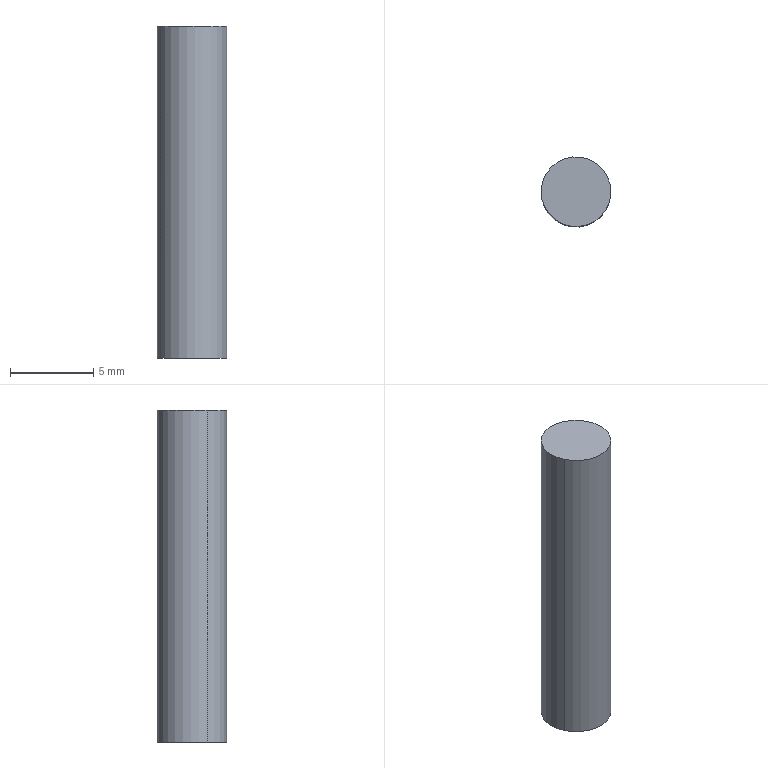Component | SolidWorks | OuterBagStorageAssembly-1_Copy_of_Part1-1 | 1 solid | 4 faces | box 4.2 x 4.2 x 20 mm | volume 277 mm3 | cylinder 2 | plane 2 | commonest cylinder face diameters 4.2 x2
build123d program:
from build123d import *

# Parameters (mm, degrees)
SKETCH1_R           = 2.1
BOSS_EXTRUDE1_DEPTH = 20


with BuildPart() as part:
    # Sketch1 → Boss-Extrude1 (new body)
    with BuildSketch(Plane.XY):
        Circle(SKETCH1_R)
    extrude(amount=BOSS_EXTRUDE1_DEPTH)


solid = part.part

# Placed as in the assembly
solid = solid.moved(Location((-354.296, 148.158, 404.536), (0, 0, 0)))
STEP:
#1=COLOUR_RGB('',0.7922,0.8196,0.9333);
#2=FILL_AREA_STYLE_COLOUR('',#1);
#3=FILL_AREA_STYLE('',(#2));
#4=SURFACE_STYLE_FILL_AREA(#3);
#5=SURFACE_SIDE_STYLE('',(#4));
#6=SURFACE_STYLE_USAGE(.BOTH.,#5);
#7=PRESENTATION_STYLE_ASSIGNMENT((#6));
#8=CARTESIAN_POINT('',(-14.023,5.797,15.927));
#9=VERTEX_POINT('',#8);
#10=CARTESIAN_POINT('',(-13.874,5.869,15.927));
#11=VERTEX_POINT('',#10);
#12=CARTESIAN_POINT('',(-13.949,5.833,15.927));
#13=DIRECTION('',(0.,0.,-1.));
#14=DIRECTION('',(-0.9002,-0.4355,0.));
#15=AXIS2_PLACEMENT_3D('',#12,#13,#14);
#16=CIRCLE('',#15,0.08268);
#17=EDGE_CURVE('',#9,#11,#16,.T.);
#18=ORIENTED_EDGE('',*,*,#17,.F.);
#19=CARTESIAN_POINT('',(-14.023,5.797,16.714));
#20=VERTEX_POINT('',#19);
#21=CARTESIAN_POINT('',(-14.023,5.797,15.927));
#22=DIRECTION('',(-0.,-0.,1.));
#23=VECTOR('',#22,39.37);
#24=LINE('',#21,#23);
#25=EDGE_CURVE('',#9,#20,#24,.T.);
#26=ORIENTED_EDGE('',*,*,#25,.T.);
#27=CARTESIAN_POINT('',(-13.874,5.869,16.714));
#28=VERTEX_POINT('',#27);
#29=CARTESIAN_POINT('',(-13.949,5.833,16.714));
#30=DIRECTION('',(0.,0.,-1.));
#31=DIRECTION('',(-0.9002,-0.4355,0.));
#32=AXIS2_PLACEMENT_3D('',#29,#30,#31);
#33=CIRCLE('',#32,0.08268);
#34=EDGE_CURVE('',#20,#28,#33,.T.);
#35=ORIENTED_EDGE('',*,*,#34,.T.);
#36=CARTESIAN_POINT('',(-13.874,5.869,15.927));
#37=DIRECTION('',(-0.,-0.,1.));
#38=VECTOR('',#37,39.37);
#39=LINE('',#36,#38);
#40=EDGE_CURVE('',#11,#28,#39,.T.);
#41=ORIENTED_EDGE('',*,*,#40,.F.);
#42=EDGE_LOOP('',(#18,#26,#35,#41));
#43=FACE_OUTER_BOUND('',#42,.T.);
#44=CARTESIAN_POINT('',(-13.949,5.833,15.927));
#45=DIRECTION('',(-0.,-0.,1.));
#46=DIRECTION('',(0.9002,0.4355,0.));
#47=AXIS2_PLACEMENT_3D('',#44,#45,#46);
#48=CYLINDRICAL_SURFACE('',#47,0.08268);
#49=ADVANCED_FACE('',(#43),#48,.T.);
#50=ORIENTED_EDGE('',*,*,#25,.F.);
#51=CARTESIAN_POINT('',(-13.949,5.833,15.927));
#52=DIRECTION('',(0.,0.,-1.));
#53=DIRECTION('',(-0.9002,-0.4355,0.));
#54=AXIS2_PLACEMENT_3D('',#51,#52,#53);
#55=CIRCLE('',#54,0.08268);
#56=EDGE_CURVE('',#11,#9,#55,.T.);
#57=ORIENTED_EDGE('',*,*,#56,.F.);
#58=ORIENTED_EDGE('',*,*,#40,.T.);
#59=CARTESIAN_POINT('',(-13.949,5.833,16.714));
#60=DIRECTION('',(0.,0.,-1.));
#61=DIRECTION('',(-0.9002,-0.4355,0.));
#62=AXIS2_PLACEMENT_3D('',#59,#60,#61);
#63=CIRCLE('',#62,0.08268);
#64=EDGE_CURVE('',#28,#20,#63,.T.);
#65=ORIENTED_EDGE('',*,*,#64,.T.);
#66=EDGE_LOOP('',(#50,#57,#58,#65));
#67=FACE_OUTER_BOUND('',#66,.T.);
#68=CARTESIAN_POINT('',(-13.949,5.833,15.927));
#69=DIRECTION('',(-0.,-0.,1.));
#70=DIRECTION('',(0.9002,0.4355,0.));
#71=AXIS2_PLACEMENT_3D('',#68,#69,#70);
#72=CYLINDRICAL_SURFACE('',#71,0.08268);
#73=ADVANCED_FACE('',(#67),#72,.T.);
#74=ORIENTED_EDGE('',*,*,#56,.T.);
#75=ORIENTED_EDGE('',*,*,#17,.T.);
#76=EDGE_LOOP('',(#74,#75));
#77=FACE_OUTER_BOUND('',#76,.T.);
#78=CARTESIAN_POINT('',(-13.949,5.833,15.927));
#79=DIRECTION('',(0.,0.,-1.));
#80=DIRECTION('',(-0.9002,-0.4355,-0.));
#81=AXIS2_PLACEMENT_3D('',#78,#79,#80);
#82=PLANE('',#81);
#83=ADVANCED_FACE('',(#77),#82,.T.);
#84=ORIENTED_EDGE('',*,*,#64,.F.);
#85=ORIENTED_EDGE('',*,*,#34,.F.);
#86=EDGE_LOOP('',(#84,#85));
#87=FACE_OUTER_BOUND('',#86,.T.);
#88=CARTESIAN_POINT('',(-13.949,5.833,16.714));
#89=DIRECTION('',(0.,0.,-1.));
#90=DIRECTION('',(-0.9002,-0.4355,-0.));
#91=AXIS2_PLACEMENT_3D('',#88,#89,#90);
#92=PLANE('',#91);
#93=ADVANCED_FACE('',(#87),#92,.F.);
#94=CLOSED_SHELL('',(#49,#73,#83,#93));
#95=MANIFOLD_SOLID_BREP('',#94);
#96=STYLED_ITEM('',(#7),#95);
#97=PRESENTATION_LAYER_ASSIGNMENT('','',(#96));
#98=CARTESIAN_POINT('',(0.,0.,0.));
#99=DIRECTION('',(0.,0.,1.));
#100=DIRECTION('',(1.,0.,0.));
#101=AXIS2_PLACEMENT_3D('',#98,#99,#100);
#102=(LENGTH_UNIT()NAMED_UNIT(*)SI_UNIT($,.METRE.));
#103=LENGTH_MEASURE_WITH_UNIT(LENGTH_MEASURE(0.0254),#102);
#104=DIMENSIONAL_EXPONENTS(1.,0.,0.,0.,0.,0.,0.);
#105=(CONVERSION_BASED_UNIT('',#103)LENGTH_UNIT()NAMED_UNIT(#104));
#106=UNCERTAINTY_MEASURE_WITH_UNIT(LENGTH_MEASURE(0.00001),#105,'','');
#107=(NAMED_UNIT(*)PLANE_ANGLE_UNIT()SI_UNIT($,.RADIAN.));
#108=(NAMED_UNIT(*)SI_UNIT($,.STERADIAN.)SOLID_ANGLE_UNIT());
#109=(GEOMETRIC_REPRESENTATION_CONTEXT(3)GLOBAL_UNCERTAINTY_ASSIGNED_CONTEXT((#106))GLOBAL_UNIT_ASSIGNED_CONTEXT((#105,#107,#108))REPRESENTATION_CONTEXT('',''));
#110=ADVANCED_BREP_SHAPE_REPRESENTATION('',(#95,#101),#109);
#111=(LENGTH_UNIT()NAMED_UNIT(*)SI_UNIT($,.METRE.));
#112=LENGTH_MEASURE_WITH_UNIT(LENGTH_MEASURE(0.0254),#111);
#113=DIMENSIONAL_EXPONENTS(1.,0.,0.,0.,0.,0.,0.);
#114=(CONVERSION_BASED_UNIT('',#112)LENGTH_UNIT()NAMED_UNIT(#113));
#115=UNCERTAINTY_MEASURE_WITH_UNIT(LENGTH_MEASURE(0.00001),#114,'','');
#116=(NAMED_UNIT(*)PLANE_ANGLE_UNIT()SI_UNIT($,.RADIAN.));
#117=(NAMED_UNIT(*)SI_UNIT($,.STERADIAN.)SOLID_ANGLE_UNIT());
#118=(GEOMETRIC_REPRESENTATION_CONTEXT(3)GLOBAL_UNCERTAINTY_ASSIGNED_CONTEXT((#115))GLOBAL_UNIT_ASSIGNED_CONTEXT((#114,#116,#117))REPRESENTATION_CONTEXT('',''));
#119=MECHANICAL_DESIGN_GEOMETRIC_PRESENTATION_REPRESENTATION('',(#96),#118);